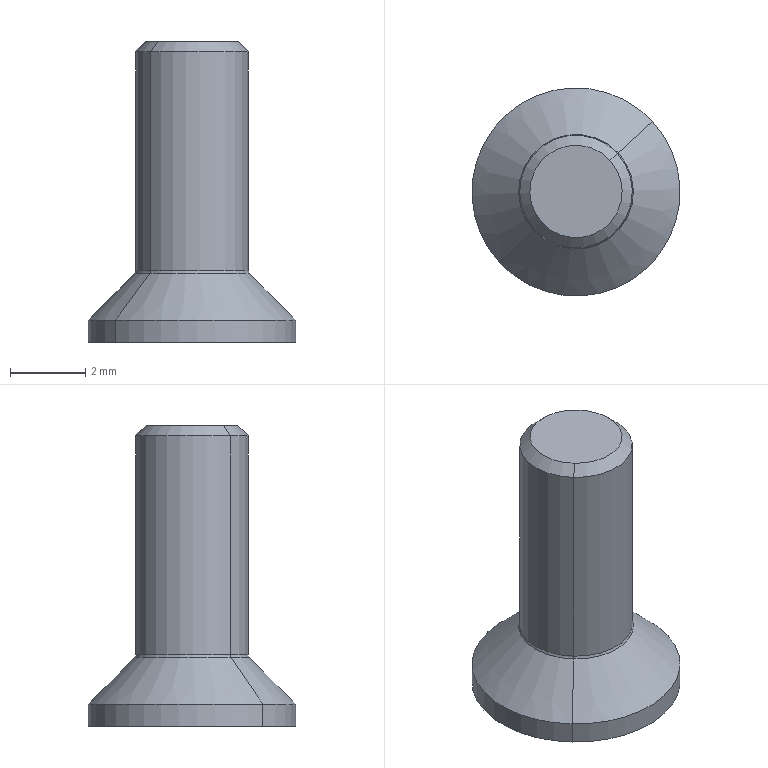Component | SolidWorks | V1ZHXTRR60SecondarySB1-1_v1ZHXTHexagon socket countersunk head screws GB_GB_FASTENER_SCREWS_HSCHS M3X8-N_1SB1-1 | 1 solid | 26 faces | box 5.54 x 5.54 x 8 mm | volume 72 mm3 | plane 14 | cone 6 | cylinder 4 | spline 2 | commonest cylinder face diameters 3 x2 5.54 x2
STEP:
#1=COLOUR_RGB('',0.7922,0.8196,0.9333);
#2=FILL_AREA_STYLE_COLOUR('',#1);
#3=FILL_AREA_STYLE('',(#2));
#4=SURFACE_STYLE_FILL_AREA(#3);
#5=SURFACE_SIDE_STYLE('',(#4));
#6=SURFACE_STYLE_USAGE(.BOTH.,#5);
#7=PRESENTATION_STYLE_ASSIGNMENT((#6));
#8=CARTESIAN_POINT('',(9.394,-8.991,18.832));
#9=VERTEX_POINT('',#8);
#10=CARTESIAN_POINT('',(9.307,-9.071,18.832));
#11=VERTEX_POINT('',#10);
#12=CARTESIAN_POINT('',(9.35,-9.031,18.832));
#13=DIRECTION('',(0.,-0.,1.));
#14=DIRECTION('',(-0.7334,-0.6798,-0.));
#15=AXIS2_PLACEMENT_3D('',#12,#13,#14);
#16=CIRCLE('',#15,0.05906);
#17=EDGE_CURVE('',#9,#11,#16,.T.);
#18=ORIENTED_EDGE('',*,*,#17,.F.);
#19=CARTESIAN_POINT('',(9.394,-8.99,18.83));
#20=VERTEX_POINT('',#19);
#21=CARTESIAN_POINT('',(9.396,-8.988,18.832));
#22=DIRECTION('',(0.6798,-0.7334,-0.));
#23=DIRECTION('',(0.7334,0.6798,0.));
#24=AXIS2_PLACEMENT_3D('',#21,#22,#23);
#25=CIRCLE('',#24,0.003937);
#26=EDGE_CURVE('',#9,#20,#25,.T.);
#27=ORIENTED_EDGE('',*,*,#26,.T.);
#28=CARTESIAN_POINT('',(9.306,-9.072,18.83));
#29=VERTEX_POINT('',#28);
#30=CARTESIAN_POINT('',(9.35,-9.031,18.83));
#31=DIRECTION('',(-0.,0.,-1.));
#32=DIRECTION('',(-0.7334,-0.6798,-0.));
#33=AXIS2_PLACEMENT_3D('',#30,#31,#32);
#34=CIRCLE('',#33,0.06021);
#35=EDGE_CURVE('',#29,#20,#34,.T.);
#36=ORIENTED_EDGE('',*,*,#35,.F.);
#37=CARTESIAN_POINT('',(9.304,-9.074,18.832));
#38=DIRECTION('',(-0.6798,0.7334,0.));
#39=DIRECTION('',(-0.7334,-0.6798,-0.));
#40=AXIS2_PLACEMENT_3D('',#37,#38,#39);
#41=CIRCLE('',#40,0.003937);
#42=EDGE_CURVE('',#11,#29,#41,.T.);
#43=ORIENTED_EDGE('',*,*,#42,.F.);
#44=EDGE_LOOP('',(#18,#27,#36,#43));
#45=FACE_OUTER_BOUND('',#44,.T.);
#46=CARTESIAN_POINT('',(9.307,-9.071,18.832));
#47=CARTESIAN_POINT('',(9.283,-9.046,18.832));
#48=CARTESIAN_POINT('',(9.285,-9.011,18.832));
#49=CARTESIAN_POINT('',(9.31,-8.988,18.832));
#50=CARTESIAN_POINT('',(9.336,-8.964,18.832));
#51=CARTESIAN_POINT('',(9.37,-8.966,18.832));
#52=CARTESIAN_POINT('',(9.394,-8.991,18.832));
#53=CARTESIAN_POINT('',(9.307,-9.071,18.831));
#54=CARTESIAN_POINT('',(9.283,-9.046,18.831));
#55=CARTESIAN_POINT('',(9.285,-9.011,18.831));
#56=CARTESIAN_POINT('',(9.31,-8.988,18.831));
#57=CARTESIAN_POINT('',(9.336,-8.964,18.831));
#58=CARTESIAN_POINT('',(9.37,-8.966,18.831));
#59=CARTESIAN_POINT('',(9.394,-8.991,18.831));
#60=CARTESIAN_POINT('',(9.307,-9.071,18.83));
#61=CARTESIAN_POINT('',(9.283,-9.046,18.83));
#62=CARTESIAN_POINT('',(9.284,-9.011,18.83));
#63=CARTESIAN_POINT('',(9.31,-8.987,18.83));
#64=CARTESIAN_POINT('',(9.335,-8.964,18.83));
#65=CARTESIAN_POINT('',(9.37,-8.965,18.83));
#66=CARTESIAN_POINT('',(9.394,-8.991,18.83));
#67=CARTESIAN_POINT('',(9.306,-9.072,18.83));
#68=CARTESIAN_POINT('',(9.282,-9.046,18.83));
#69=CARTESIAN_POINT('',(9.283,-9.011,18.83));
#70=CARTESIAN_POINT('',(9.309,-8.987,18.83));
#71=CARTESIAN_POINT('',(9.335,-8.963,18.83));
#72=CARTESIAN_POINT('',(9.37,-8.964,18.83));
#73=CARTESIAN_POINT('',(9.394,-8.99,18.83));
#74=(BOUNDED_SURFACE()B_SPLINE_SURFACE(3,3,((#46,#47,#48,#49,#50,#51,#52),(#53,#54,#55,#56,#57,#58,#59),(#60,#61,#62,#63,#64,#65,#66),(#67,#68,#69,#70,#71,#72,#73)),.UNSPECIFIED.,.F.,.F.,.F.)B_SPLINE_SURFACE_WITH_KNOTS((4,4),(4,3,4),(0.,1.),(0.,0.5,1.),.UNSPECIFIED.)GEOMETRIC_REPRESENTATION_ITEM()RATIONAL_B_SPLINE_SURFACE(((1.,0.8047,0.8047,1.,0.8047,0.8047,1.),(0.9493,0.7639,0.7639,0.9493,0.7639,0.7639,0.9493),(0.9493,0.7639,0.7639,0.9493,0.7639,0.7639,0.9493),(1.,0.8047,0.8047,1.,0.8047,0.8047,1.)))REPRESENTATION_ITEM('')SURFACE());
#75=ADVANCED_FACE('',(#45),#74,.F.);
#76=CARTESIAN_POINT('',(9.307,-9.071,19.062));
#77=VERTEX_POINT('',#76);
#78=CARTESIAN_POINT('',(9.394,-8.991,19.062));
#79=VERTEX_POINT('',#78);
#80=CARTESIAN_POINT('',(9.35,-9.031,19.062));
#81=DIRECTION('',(-0.,0.,-1.));
#82=DIRECTION('',(-0.7334,-0.6798,-0.));
#83=AXIS2_PLACEMENT_3D('',#80,#81,#82);
#84=CIRCLE('',#83,0.05906);
#85=EDGE_CURVE('',#77,#79,#84,.T.);
#86=ORIENTED_EDGE('',*,*,#85,.T.);
#87=CARTESIAN_POINT('',(9.394,-8.991,18.734));
#88=DIRECTION('',(-0.,0.,-1.));
#89=VECTOR('',#88,39.37);
#90=LINE('',#87,#89);
#91=EDGE_CURVE('',#79,#9,#90,.T.);
#92=ORIENTED_EDGE('',*,*,#91,.T.);
#93=ORIENTED_EDGE('',*,*,#17,.T.);
#94=CARTESIAN_POINT('',(9.307,-9.071,18.734));
#95=DIRECTION('',(-0.,0.,-1.));
#96=VECTOR('',#95,39.37);
#97=LINE('',#94,#96);
#98=EDGE_CURVE('',#77,#11,#97,.T.);
#99=ORIENTED_EDGE('',*,*,#98,.F.);
#100=EDGE_LOOP('',(#86,#92,#93,#99));
#101=FACE_OUTER_BOUND('',#100,.T.);
#102=CARTESIAN_POINT('',(9.35,-9.031,18.734));
#103=DIRECTION('',(-0.,0.,-1.));
#104=DIRECTION('',(-0.7334,-0.6798,-0.));
#105=AXIS2_PLACEMENT_3D('',#102,#103,#104);
#106=CYLINDRICAL_SURFACE('',#105,0.05906);
#107=ADVANCED_FACE('',(#101),#106,.T.);
#108=CARTESIAN_POINT('',(9.315,-9.064,19.072));
#109=VERTEX_POINT('',#108);
#110=CARTESIAN_POINT('',(9.386,-8.998,19.072));
#111=VERTEX_POINT('',#110);
#112=CARTESIAN_POINT('',(9.35,-9.031,19.072));
#113=DIRECTION('',(-0.,0.,-1.));
#114=DIRECTION('',(-0.7334,-0.6798,-0.));
#115=AXIS2_PLACEMENT_3D('',#112,#113,#114);
#116=CIRCLE('',#115,0.04841);
#117=EDGE_CURVE('',#109,#111,#116,.T.);
#118=ORIENTED_EDGE('',*,*,#117,.T.);
#119=CARTESIAN_POINT('',(9.394,-8.991,19.062));
#120=DIRECTION('',(0.5186,0.4807,-0.7071));
#121=VECTOR('',#120,39.37);
#122=LINE('',#119,#121);
#123=EDGE_CURVE('',#111,#79,#122,.T.);
#124=ORIENTED_EDGE('',*,*,#123,.T.);
#125=ORIENTED_EDGE('',*,*,#85,.F.);
#126=CARTESIAN_POINT('',(9.307,-9.071,19.062));
#127=DIRECTION('',(-0.5186,-0.4807,-0.7071));
#128=VECTOR('',#127,39.37);
#129=LINE('',#126,#128);
#130=EDGE_CURVE('',#109,#77,#129,.T.);
#131=ORIENTED_EDGE('',*,*,#130,.F.);
#132=EDGE_LOOP('',(#118,#124,#125,#131));
#133=FACE_OUTER_BOUND('',#132,.T.);
#134=CARTESIAN_POINT('',(9.35,-9.031,19.062));
#135=DIRECTION('',(-0.,0.,-1.));
#136=DIRECTION('',(-0.7334,-0.6798,-0.));
#137=AXIS2_PLACEMENT_3D('',#134,#135,#136);
#138=CONICAL_SURFACE('',#137,0.05906,0.7854);
#139=ADVANCED_FACE('',(#133),#138,.T.);
#140=ORIENTED_EDGE('',*,*,#35,.T.);
#141=CARTESIAN_POINT('',(9.43,-8.957,18.781));
#142=VERTEX_POINT('',#141);
#143=CARTESIAN_POINT('',(9.43,-8.957,18.781));
#144=DIRECTION('',(0.5186,0.4807,-0.7071));
#145=VECTOR('',#144,39.37);
#146=LINE('',#143,#145);
#147=EDGE_CURVE('',#20,#142,#146,.T.);
#148=ORIENTED_EDGE('',*,*,#147,.T.);
#149=CARTESIAN_POINT('',(9.27,-9.105,18.781));
#150=VERTEX_POINT('',#149);
#151=CARTESIAN_POINT('',(9.35,-9.031,18.781));
#152=DIRECTION('',(0.,-0.,1.));
#153=DIRECTION('',(-0.7334,-0.6798,-0.));
#154=AXIS2_PLACEMENT_3D('',#151,#152,#153);
#155=CIRCLE('',#154,0.1091);
#156=EDGE_CURVE('',#142,#150,#155,.T.);
#157=ORIENTED_EDGE('',*,*,#156,.T.);
#158=CARTESIAN_POINT('',(9.27,-9.105,18.781));
#159=DIRECTION('',(-0.5186,-0.4807,-0.7071));
#160=VECTOR('',#159,39.37);
#161=LINE('',#158,#160);
#162=EDGE_CURVE('',#29,#150,#161,.T.);
#163=ORIENTED_EDGE('',*,*,#162,.F.);
#164=EDGE_LOOP('',(#140,#148,#157,#163));
#165=FACE_OUTER_BOUND('',#164,.T.);
#166=CARTESIAN_POINT('',(9.35,-9.031,18.781));
#167=DIRECTION('',(-0.,0.,-1.));
#168=DIRECTION('',(-0.7334,-0.6798,-0.));
#169=AXIS2_PLACEMENT_3D('',#166,#167,#168);
#170=CONICAL_SURFACE('',#169,0.1091,0.7854);
#171=ADVANCED_FACE('',(#165),#170,.T.);
#172=CARTESIAN_POINT('',(9.43,-8.957,18.757));
#173=VERTEX_POINT('',#172);
#174=CARTESIAN_POINT('',(9.27,-9.105,18.757));
#175=VERTEX_POINT('',#174);
#176=CARTESIAN_POINT('',(9.35,-9.031,18.757));
#177=DIRECTION('',(0.,-0.,1.));
#178=DIRECTION('',(0.7334,0.6798,0.));
#179=AXIS2_PLACEMENT_3D('',#176,#177,#178);
#180=CIRCLE('',#179,0.1091);
#181=EDGE_CURVE('',#173,#175,#180,.T.);
#182=ORIENTED_EDGE('',*,*,#181,.T.);
#183=CARTESIAN_POINT('',(9.27,-9.105,19.224));
#184=DIRECTION('',(0.,-0.,1.));
#185=VECTOR('',#184,39.37);
#186=LINE('',#183,#185);
#187=EDGE_CURVE('',#175,#150,#186,.T.);
#188=ORIENTED_EDGE('',*,*,#187,.T.);
#189=ORIENTED_EDGE('',*,*,#156,.F.);
#190=CARTESIAN_POINT('',(9.43,-8.957,19.224));
#191=DIRECTION('',(0.,-0.,1.));
#192=VECTOR('',#191,39.37);
#193=LINE('',#190,#192);
#194=EDGE_CURVE('',#173,#142,#193,.T.);
#195=ORIENTED_EDGE('',*,*,#194,.F.);
#196=EDGE_LOOP('',(#182,#188,#189,#195));
#197=FACE_OUTER_BOUND('',#196,.T.);
#198=CARTESIAN_POINT('',(9.35,-9.031,19.224));
#199=DIRECTION('',(0.,-0.,1.));
#200=DIRECTION('',(0.7334,0.6798,0.));
#201=AXIS2_PLACEMENT_3D('',#198,#199,#200);
#202=CYLINDRICAL_SURFACE('',#201,0.1091);
#203=ADVANCED_FACE('',(#197),#202,.T.);
#204=CARTESIAN_POINT('',(9.35,-9.031,18.823));
#205=VERTEX_POINT('',#204);
#206=CARTESIAN_POINT('',(9.321,-9.058,18.801));
#207=VERTEX_POINT('',#206);
#208=CARTESIAN_POINT('',(9.321,-9.058,18.801));
#209=DIRECTION('',(-0.6351,-0.5888,-0.5));
#210=VECTOR('',#209,39.37);
#211=LINE('',#208,#210);
#212=EDGE_CURVE('',#205,#207,#211,.T.);
#213=ORIENTED_EDGE('',*,*,#212,.F.);
#214=CARTESIAN_POINT('',(9.379,-9.004,18.801));
#215=VERTEX_POINT('',#214);
#216=CARTESIAN_POINT('',(9.379,-9.004,18.801));
#217=DIRECTION('',(0.6351,0.5888,-0.5));
#218=VECTOR('',#217,39.37);
#219=LINE('',#216,#218);
#220=EDGE_CURVE('',#205,#215,#219,.T.);
#221=ORIENTED_EDGE('',*,*,#220,.T.);
#222=CARTESIAN_POINT('',(9.389,-9.022,18.801));
#223=VERTEX_POINT('',#222);
#224=CARTESIAN_POINT('',(9.35,-9.031,18.801));
#225=DIRECTION('',(-0.,0.,-1.));
#226=DIRECTION('',(-0.7334,-0.6798,-0.));
#227=AXIS2_PLACEMENT_3D('',#224,#225,#226);
#228=CIRCLE('',#227,0.03937);
#229=EDGE_CURVE('',#215,#223,#228,.T.);
#230=ORIENTED_EDGE('',*,*,#229,.T.);
#231=CARTESIAN_POINT('',(9.377,-9.06,18.801));
#232=VERTEX_POINT('',#231);
#233=CARTESIAN_POINT('',(9.35,-9.031,18.801));
#234=DIRECTION('',(-0.,0.,-1.));
#235=DIRECTION('',(-0.7334,-0.6798,-0.));
#236=AXIS2_PLACEMENT_3D('',#233,#234,#235);
#237=CIRCLE('',#236,0.03937);
#238=EDGE_CURVE('',#223,#232,#237,.T.);
#239=ORIENTED_EDGE('',*,*,#238,.T.);
#240=CARTESIAN_POINT('',(9.339,-9.069,18.801));
#241=VERTEX_POINT('',#240);
#242=CARTESIAN_POINT('',(9.35,-9.031,18.801));
#243=DIRECTION('',(-0.,0.,-1.));
#244=DIRECTION('',(-0.7334,-0.6798,-0.));
#245=AXIS2_PLACEMENT_3D('',#242,#243,#244);
#246=CIRCLE('',#245,0.03937);
#247=EDGE_CURVE('',#232,#241,#246,.T.);
#248=ORIENTED_EDGE('',*,*,#247,.T.);
#249=CARTESIAN_POINT('',(9.35,-9.031,18.801));
#250=DIRECTION('',(-0.,0.,-1.));
#251=DIRECTION('',(-0.7334,-0.6798,-0.));
#252=AXIS2_PLACEMENT_3D('',#249,#250,#251);
#253=CIRCLE('',#252,0.03937);
#254=EDGE_CURVE('',#241,#207,#253,.T.);
#255=ORIENTED_EDGE('',*,*,#254,.T.);
#256=EDGE_LOOP('',(#213,#221,#230,#239,#248,#255));
#257=FACE_OUTER_BOUND('',#256,.T.);
#258=CARTESIAN_POINT('',(9.35,-9.031,18.801));
#259=DIRECTION('',(-0.,0.,-1.));
#260=DIRECTION('',(-0.7334,-0.6798,-0.));
#261=AXIS2_PLACEMENT_3D('',#258,#259,#260);
#262=CONICAL_SURFACE('',#261,0.03937,1.047);
#263=ADVANCED_FACE('',(#257),#262,.F.);
#264=ORIENTED_EDGE('',*,*,#91,.F.);
#265=CARTESIAN_POINT('',(9.35,-9.031,19.062));
#266=DIRECTION('',(-0.,0.,-1.));
#267=DIRECTION('',(-0.7334,-0.6798,-0.));
#268=AXIS2_PLACEMENT_3D('',#265,#266,#267);
#269=CIRCLE('',#268,0.05906);
#270=EDGE_CURVE('',#79,#77,#269,.T.);
#271=ORIENTED_EDGE('',*,*,#270,.T.);
#272=ORIENTED_EDGE('',*,*,#98,.T.);
#273=CARTESIAN_POINT('',(9.35,-9.031,18.832));
#274=DIRECTION('',(0.,-0.,1.));
#275=DIRECTION('',(-0.7334,-0.6798,-0.));
#276=AXIS2_PLACEMENT_3D('',#273,#274,#275);
#277=CIRCLE('',#276,0.05906);
#278=EDGE_CURVE('',#11,#9,#277,.T.);
#279=ORIENTED_EDGE('',*,*,#278,.T.);
#280=EDGE_LOOP('',(#264,#271,#272,#279));
#281=FACE_OUTER_BOUND('',#280,.T.);
#282=CARTESIAN_POINT('',(9.35,-9.031,18.734));
#283=DIRECTION('',(-0.,0.,-1.));
#284=DIRECTION('',(-0.7334,-0.6798,-0.));
#285=AXIS2_PLACEMENT_3D('',#282,#283,#284);
#286=CYLINDRICAL_SURFACE('',#285,0.05906);
#287=ADVANCED_FACE('',(#281),#286,.T.);
#288=ORIENTED_EDGE('',*,*,#26,.F.);
#289=ORIENTED_EDGE('',*,*,#278,.F.);
#290=ORIENTED_EDGE('',*,*,#42,.T.);
#291=CARTESIAN_POINT('',(9.35,-9.031,18.83));
#292=DIRECTION('',(-0.,0.,-1.));
#293=DIRECTION('',(-0.7334,-0.6798,-0.));
#294=AXIS2_PLACEMENT_3D('',#291,#292,#293);
#295=CIRCLE('',#294,0.06021);
#296=EDGE_CURVE('',#20,#29,#295,.T.);
#297=ORIENTED_EDGE('',*,*,#296,.F.);
#298=EDGE_LOOP('',(#288,#289,#290,#297));
#299=FACE_OUTER_BOUND('',#298,.T.);
#300=CARTESIAN_POINT('',(9.394,-8.991,18.832));
#301=CARTESIAN_POINT('',(9.474,-9.078,18.832));
#302=CARTESIAN_POINT('',(9.387,-9.158,18.832));
#303=CARTESIAN_POINT('',(9.307,-9.071,18.832));
#304=CARTESIAN_POINT('',(9.394,-8.991,18.831));
#305=CARTESIAN_POINT('',(9.474,-9.078,18.831));
#306=CARTESIAN_POINT('',(9.387,-9.158,18.831));
#307=CARTESIAN_POINT('',(9.307,-9.071,18.831));
#308=CARTESIAN_POINT('',(9.394,-8.991,18.83));
#309=CARTESIAN_POINT('',(9.475,-9.078,18.83));
#310=CARTESIAN_POINT('',(9.388,-9.159,18.83));
#311=CARTESIAN_POINT('',(9.307,-9.071,18.83));
#312=CARTESIAN_POINT('',(9.394,-8.99,18.83));
#313=CARTESIAN_POINT('',(9.476,-9.078,18.83));
#314=CARTESIAN_POINT('',(9.388,-9.16,18.83));
#315=CARTESIAN_POINT('',(9.306,-9.072,18.83));
#316=(BOUNDED_SURFACE()B_SPLINE_SURFACE(3,3,((#300,#301,#302,#303),(#304,#305,#306,#307),(#308,#309,#310,#311),(#312,#313,#314,#315)),.UNSPECIFIED.,.F.,.F.,.F.)B_SPLINE_SURFACE_WITH_KNOTS((4,4),(4,4),(0.,1.),(0.,1.),.UNSPECIFIED.)GEOMETRIC_REPRESENTATION_ITEM()RATIONAL_B_SPLINE_SURFACE(((1.,0.3333,0.3333,1.),(0.9493,0.3164,0.3164,0.9493),(0.9493,0.3164,0.3164,0.9493),(1.,0.3333,0.3333,1.)))REPRESENTATION_ITEM('')SURFACE());
#317=ADVANCED_FACE('',(#299),#316,.F.);
#318=ORIENTED_EDGE('',*,*,#123,.F.);
#319=CARTESIAN_POINT('',(9.35,-9.031,19.072));
#320=DIRECTION('',(-0.,0.,-1.));
#321=DIRECTION('',(-0.7334,-0.6798,-0.));
#322=AXIS2_PLACEMENT_3D('',#319,#320,#321);
#323=CIRCLE('',#322,0.04841);
#324=EDGE_CURVE('',#111,#109,#323,.T.);
#325=ORIENTED_EDGE('',*,*,#324,.T.);
#326=ORIENTED_EDGE('',*,*,#130,.T.);
#327=ORIENTED_EDGE('',*,*,#270,.F.);
#328=EDGE_LOOP('',(#318,#325,#326,#327));
#329=FACE_OUTER_BOUND('',#328,.T.);
#330=CARTESIAN_POINT('',(9.35,-9.031,19.062));
#331=DIRECTION('',(-0.,0.,-1.));
#332=DIRECTION('',(-0.7334,-0.6798,-0.));
#333=AXIS2_PLACEMENT_3D('',#330,#331,#332);
#334=CONICAL_SURFACE('',#333,0.05906,0.7854);
#335=ADVANCED_FACE('',(#329),#334,.T.);
#336=ORIENTED_EDGE('',*,*,#147,.F.);
#337=ORIENTED_EDGE('',*,*,#296,.T.);
#338=ORIENTED_EDGE('',*,*,#162,.T.);
#339=CARTESIAN_POINT('',(9.35,-9.031,18.781));
#340=DIRECTION('',(0.,-0.,1.));
#341=DIRECTION('',(-0.7334,-0.6798,-0.));
#342=AXIS2_PLACEMENT_3D('',#339,#340,#341);
#343=CIRCLE('',#342,0.1091);
#344=EDGE_CURVE('',#150,#142,#343,.T.);
#345=ORIENTED_EDGE('',*,*,#344,.T.);
#346=EDGE_LOOP('',(#336,#337,#338,#345));
#347=FACE_OUTER_BOUND('',#346,.T.);
#348=CARTESIAN_POINT('',(9.35,-9.031,18.781));
#349=DIRECTION('',(-0.,0.,-1.));
#350=DIRECTION('',(-0.7334,-0.6798,-0.));
#351=AXIS2_PLACEMENT_3D('',#348,#349,#350);
#352=CONICAL_SURFACE('',#351,0.1091,0.7854);
#353=ADVANCED_FACE('',(#347),#352,.T.);
#354=ORIENTED_EDGE('',*,*,#117,.F.);
#355=ORIENTED_EDGE('',*,*,#324,.F.);
#356=EDGE_LOOP('',(#354,#355));
#357=FACE_OUTER_BOUND('',#356,.T.);
#358=CARTESIAN_POINT('',(9.31,-8.988,19.072));
#359=DIRECTION('',(-0.,0.,-1.));
#360=DIRECTION('',(-0.7334,-0.6798,-0.));
#361=AXIS2_PLACEMENT_3D('',#358,#359,#360);
#362=PLANE('',#361);
#363=ADVANCED_FACE('',(#357),#362,.F.);
#364=ORIENTED_EDGE('',*,*,#187,.F.);
#365=CARTESIAN_POINT('',(9.35,-9.031,18.757));
#366=DIRECTION('',(0.,-0.,1.));
#367=DIRECTION('',(0.7334,0.6798,0.));
#368=AXIS2_PLACEMENT_3D('',#365,#366,#367);
#369=CIRCLE('',#368,0.1091);
#370=EDGE_CURVE('',#175,#173,#369,.T.);
#371=ORIENTED_EDGE('',*,*,#370,.T.);
#372=ORIENTED_EDGE('',*,*,#194,.T.);
#373=ORIENTED_EDGE('',*,*,#344,.F.);
#374=EDGE_LOOP('',(#364,#371,#372,#373));
#375=FACE_OUTER_BOUND('',#374,.T.);
#376=CARTESIAN_POINT('',(9.35,-9.031,19.224));
#377=DIRECTION('',(0.,-0.,1.));
#378=DIRECTION('',(0.7334,0.6798,0.));
#379=AXIS2_PLACEMENT_3D('',#376,#377,#378);
#380=CYLINDRICAL_SURFACE('',#379,0.1091);
#381=ADVANCED_FACE('',(#375),#380,.T.);
#382=CARTESIAN_POINT('',(9.34,-8.987,18.757));
#383=VERTEX_POINT('',#382);
#384=CARTESIAN_POINT('',(9.384,-9.,18.757));
#385=VERTEX_POINT('',#384);
#386=CARTESIAN_POINT('',(9.34,-8.987,18.757));
#387=DIRECTION('',(0.9554,-0.2952,-0.));
#388=VECTOR('',#387,39.37);
#389=LINE('',#386,#388);
#390=EDGE_CURVE('',#383,#385,#389,.T.);
#391=ORIENTED_EDGE('',*,*,#390,.F.);
#392=CARTESIAN_POINT('',(9.307,-9.018,18.757));
#393=VERTEX_POINT('',#392);
#394=CARTESIAN_POINT('',(9.324,-9.002,18.757));
#395=DIRECTION('',(0.7334,0.6798,0.));
#396=VECTOR('',#395,39.37);
#397=LINE('',#394,#396);
#398=EDGE_CURVE('',#393,#383,#397,.T.);
#399=ORIENTED_EDGE('',*,*,#398,.F.);
#400=CARTESIAN_POINT('',(9.317,-9.062,18.757));
#401=VERTEX_POINT('',#400);
#402=CARTESIAN_POINT('',(9.317,-9.062,18.757));
#403=DIRECTION('',(-0.2221,0.975,0.));
#404=VECTOR('',#403,39.37);
#405=LINE('',#402,#404);
#406=EDGE_CURVE('',#401,#393,#405,.T.);
#407=ORIENTED_EDGE('',*,*,#406,.F.);
#408=CARTESIAN_POINT('',(9.36,-9.075,18.757));
#409=VERTEX_POINT('',#408);
#410=CARTESIAN_POINT('',(9.36,-9.075,18.757));
#411=DIRECTION('',(-0.9554,0.2952,0.));
#412=VECTOR('',#411,39.37);
#413=LINE('',#410,#412);
#414=EDGE_CURVE('',#409,#401,#413,.T.);
#415=ORIENTED_EDGE('',*,*,#414,.F.);
#416=CARTESIAN_POINT('',(9.394,-9.044,18.757));
#417=VERTEX_POINT('',#416);
#418=CARTESIAN_POINT('',(9.377,-9.06,18.757));
#419=DIRECTION('',(-0.7334,-0.6798,-0.));
#420=VECTOR('',#419,39.37);
#421=LINE('',#418,#420);
#422=EDGE_CURVE('',#417,#409,#421,.T.);
#423=ORIENTED_EDGE('',*,*,#422,.F.);
#424=CARTESIAN_POINT('',(9.384,-9.,18.757));
#425=DIRECTION('',(0.2221,-0.975,-0.));
#426=VECTOR('',#425,39.37);
#427=LINE('',#424,#426);
#428=EDGE_CURVE('',#385,#417,#427,.T.);
#429=ORIENTED_EDGE('',*,*,#428,.F.);
#430=EDGE_LOOP('',(#391,#399,#407,#415,#423,#429));
#431=FACE_BOUND('',#430,.T.);
#432=ORIENTED_EDGE('',*,*,#181,.F.);
#433=ORIENTED_EDGE('',*,*,#370,.F.);
#434=EDGE_LOOP('',(#432,#433));
#435=FACE_OUTER_BOUND('',#434,.T.);
#436=CARTESIAN_POINT('',(9.35,-9.031,18.757));
#437=DIRECTION('',(0.,-0.,1.));
#438=DIRECTION('',(0.7334,0.6798,0.));
#439=AXIS2_PLACEMENT_3D('',#436,#437,#438);
#440=PLANE('',#439);
#441=ADVANCED_FACE('',(#431,#435),#440,.F.);
#442=CARTESIAN_POINT('',(9.384,-9.,18.801));
#443=VERTEX_POINT('',#442);
#444=CARTESIAN_POINT('',(9.394,-9.044,18.801));
#445=DIRECTION('',(-0.2221,0.975,0.));
#446=VECTOR('',#445,39.37);
#447=LINE('',#444,#446);
#448=EDGE_CURVE('',#223,#443,#447,.T.);
#449=ORIENTED_EDGE('',*,*,#448,.T.);
#450=CARTESIAN_POINT('',(9.384,-9.,18.801));
#451=DIRECTION('',(-0.,0.,-1.));
#452=VECTOR('',#451,39.37);
#453=LINE('',#450,#452);
#454=EDGE_CURVE('',#443,#385,#453,.T.);
#455=ORIENTED_EDGE('',*,*,#454,.T.);
#456=ORIENTED_EDGE('',*,*,#428,.T.);
#457=CARTESIAN_POINT('',(9.394,-9.044,18.801));
#458=VERTEX_POINT('',#457);
#459=CARTESIAN_POINT('',(9.394,-9.044,18.801));
#460=DIRECTION('',(0.,-0.,1.));
#461=VECTOR('',#460,39.37);
#462=LINE('',#459,#461);
#463=EDGE_CURVE('',#417,#458,#462,.T.);
#464=ORIENTED_EDGE('',*,*,#463,.T.);
#465=CARTESIAN_POINT('',(9.394,-9.044,18.801));
#466=DIRECTION('',(-0.2221,0.975,0.));
#467=VECTOR('',#466,39.37);
#468=LINE('',#465,#467);
#469=EDGE_CURVE('',#458,#223,#468,.T.);
#470=ORIENTED_EDGE('',*,*,#469,.T.);
#471=EDGE_LOOP('',(#449,#455,#456,#464,#470));
#472=FACE_OUTER_BOUND('',#471,.T.);
#473=CARTESIAN_POINT('',(9.394,-9.044,18.801));
#474=DIRECTION('',(-0.975,-0.2221,-0.));
#475=DIRECTION('',(0.2221,-0.975,-0.));
#476=AXIS2_PLACEMENT_3D('',#473,#474,#475);
#477=PLANE('',#476);
#478=ADVANCED_FACE('',(#472),#477,.T.);
#479=CARTESIAN_POINT('',(9.362,-8.993,18.801));
#480=VERTEX_POINT('',#479);
#481=CARTESIAN_POINT('',(9.34,-8.987,18.801));
#482=VERTEX_POINT('',#481);
#483=CARTESIAN_POINT('',(9.384,-9.,18.801));
#484=DIRECTION('',(-0.9554,0.2952,0.));
#485=VECTOR('',#484,39.37);
#486=LINE('',#483,#485);
#487=EDGE_CURVE('',#480,#482,#486,.T.);
#488=ORIENTED_EDGE('',*,*,#487,.T.);
#489=CARTESIAN_POINT('',(9.34,-8.987,18.801));
#490=DIRECTION('',(-0.,0.,-1.));
#491=VECTOR('',#490,39.37);
#492=LINE('',#489,#491);
#493=EDGE_CURVE('',#482,#383,#492,.T.);
#494=ORIENTED_EDGE('',*,*,#493,.T.);
#495=ORIENTED_EDGE('',*,*,#390,.T.);
#496=ORIENTED_EDGE('',*,*,#454,.F.);
#497=CARTESIAN_POINT('',(9.384,-9.,18.801));
#498=DIRECTION('',(-0.9554,0.2952,0.));
#499=VECTOR('',#498,39.37);
#500=LINE('',#497,#499);
#501=EDGE_CURVE('',#443,#480,#500,.T.);
#502=ORIENTED_EDGE('',*,*,#501,.T.);
#503=EDGE_LOOP('',(#488,#494,#495,#496,#502));
#504=FACE_OUTER_BOUND('',#503,.T.);
#505=CARTESIAN_POINT('',(9.384,-9.,18.801));
#506=DIRECTION('',(-0.2952,-0.9554,-0.));
#507=DIRECTION('',(0.9554,-0.2952,-0.));
#508=AXIS2_PLACEMENT_3D('',#505,#506,#507);
#509=PLANE('',#508);
#510=ADVANCED_FACE('',(#504),#509,.T.);
#511=CARTESIAN_POINT('',(9.324,-9.002,18.801));
#512=VERTEX_POINT('',#511);
#513=CARTESIAN_POINT('',(9.307,-9.018,18.801));
#514=VERTEX_POINT('',#513);
#515=CARTESIAN_POINT('',(9.34,-8.987,18.801));
#516=DIRECTION('',(-0.7334,-0.6798,-0.));
#517=VECTOR('',#516,39.37);
#518=LINE('',#515,#517);
#519=EDGE_CURVE('',#512,#514,#518,.T.);
#520=ORIENTED_EDGE('',*,*,#519,.T.);
#521=CARTESIAN_POINT('',(9.307,-9.018,18.801));
#522=DIRECTION('',(-0.,0.,-1.));
#523=VECTOR('',#522,39.37);
#524=LINE('',#521,#523);
#525=EDGE_CURVE('',#514,#393,#524,.T.);
#526=ORIENTED_EDGE('',*,*,#525,.T.);
#527=ORIENTED_EDGE('',*,*,#398,.T.);
#528=ORIENTED_EDGE('',*,*,#493,.F.);
#529=CARTESIAN_POINT('',(9.34,-8.987,18.801));
#530=DIRECTION('',(-0.7334,-0.6798,-0.));
#531=VECTOR('',#530,39.37);
#532=LINE('',#529,#531);
#533=EDGE_CURVE('',#482,#512,#532,.T.);
#534=ORIENTED_EDGE('',*,*,#533,.T.);
#535=EDGE_LOOP('',(#520,#526,#527,#528,#534));
#536=FACE_OUTER_BOUND('',#535,.T.);
#537=CARTESIAN_POINT('',(9.34,-8.987,18.801));
#538=DIRECTION('',(0.6798,-0.7334,-0.));
#539=DIRECTION('',(0.7334,0.6798,0.));
#540=AXIS2_PLACEMENT_3D('',#537,#538,#539);
#541=PLANE('',#540);
#542=ADVANCED_FACE('',(#536),#541,.T.);
#543=CARTESIAN_POINT('',(9.312,-9.04,18.801));
#544=VERTEX_POINT('',#543);
#545=CARTESIAN_POINT('',(9.317,-9.062,18.801));
#546=VERTEX_POINT('',#545);
#547=CARTESIAN_POINT('',(9.307,-9.018,18.801));
#548=DIRECTION('',(0.2221,-0.975,-0.));
#549=VECTOR('',#548,39.37);
#550=LINE('',#547,#549);
#551=EDGE_CURVE('',#544,#546,#550,.T.);
#552=ORIENTED_EDGE('',*,*,#551,.T.);
#553=CARTESIAN_POINT('',(9.317,-9.062,18.801));
#554=DIRECTION('',(-0.,0.,-1.));
#555=VECTOR('',#554,39.37);
#556=LINE('',#553,#555);
#557=EDGE_CURVE('',#546,#401,#556,.T.);
#558=ORIENTED_EDGE('',*,*,#557,.T.);
#559=ORIENTED_EDGE('',*,*,#406,.T.);
#560=ORIENTED_EDGE('',*,*,#525,.F.);
#561=CARTESIAN_POINT('',(9.307,-9.018,18.801));
#562=DIRECTION('',(0.2221,-0.975,-0.));
#563=VECTOR('',#562,39.37);
#564=LINE('',#561,#563);
#565=EDGE_CURVE('',#514,#544,#564,.T.);
#566=ORIENTED_EDGE('',*,*,#565,.T.);
#567=EDGE_LOOP('',(#552,#558,#559,#560,#566));
#568=FACE_OUTER_BOUND('',#567,.T.);
#569=CARTESIAN_POINT('',(9.307,-9.018,18.801));
#570=DIRECTION('',(0.975,0.2221,0.));
#571=DIRECTION('',(-0.2221,0.975,0.));
#572=AXIS2_PLACEMENT_3D('',#569,#570,#571);
#573=PLANE('',#572);
#574=ADVANCED_FACE('',(#568),#573,.T.);
#575=CARTESIAN_POINT('',(9.36,-9.075,18.801));
#576=VERTEX_POINT('',#575);
#577=CARTESIAN_POINT('',(9.317,-9.062,18.801));
#578=DIRECTION('',(0.9554,-0.2952,-0.));
#579=VECTOR('',#578,39.37);
#580=LINE('',#577,#579);
#581=EDGE_CURVE('',#241,#576,#580,.T.);
#582=ORIENTED_EDGE('',*,*,#581,.T.);
#583=CARTESIAN_POINT('',(9.36,-9.075,18.801));
#584=DIRECTION('',(-0.,0.,-1.));
#585=VECTOR('',#584,39.37);
#586=LINE('',#583,#585);
#587=EDGE_CURVE('',#576,#409,#586,.T.);
#588=ORIENTED_EDGE('',*,*,#587,.T.);
#589=ORIENTED_EDGE('',*,*,#414,.T.);
#590=ORIENTED_EDGE('',*,*,#557,.F.);
#591=CARTESIAN_POINT('',(9.317,-9.062,18.801));
#592=DIRECTION('',(0.9554,-0.2952,-0.));
#593=VECTOR('',#592,39.37);
#594=LINE('',#591,#593);
#595=EDGE_CURVE('',#546,#241,#594,.T.);
#596=ORIENTED_EDGE('',*,*,#595,.T.);
#597=EDGE_LOOP('',(#582,#588,#589,#590,#596));
#598=FACE_OUTER_BOUND('',#597,.T.);
#599=CARTESIAN_POINT('',(9.317,-9.062,18.801));
#600=DIRECTION('',(0.2952,0.9554,0.));
#601=DIRECTION('',(-0.9554,0.2952,0.));
#602=AXIS2_PLACEMENT_3D('',#599,#600,#601);
#603=PLANE('',#602);
#604=ADVANCED_FACE('',(#598),#603,.T.);
#605=CARTESIAN_POINT('',(9.36,-9.075,18.801));
#606=DIRECTION('',(0.7334,0.6798,0.));
#607=VECTOR('',#606,39.37);
#608=LINE('',#605,#607);
#609=EDGE_CURVE('',#232,#458,#608,.T.);
#610=ORIENTED_EDGE('',*,*,#609,.T.);
#611=ORIENTED_EDGE('',*,*,#463,.F.);
#612=ORIENTED_EDGE('',*,*,#422,.T.);
#613=ORIENTED_EDGE('',*,*,#587,.F.);
#614=CARTESIAN_POINT('',(9.36,-9.075,18.801));
#615=DIRECTION('',(0.7334,0.6798,0.));
#616=VECTOR('',#615,39.37);
#617=LINE('',#614,#616);
#618=EDGE_CURVE('',#576,#232,#617,.T.);
#619=ORIENTED_EDGE('',*,*,#618,.T.);
#620=EDGE_LOOP('',(#610,#611,#612,#613,#619));
#621=FACE_OUTER_BOUND('',#620,.T.);
#622=CARTESIAN_POINT('',(9.36,-9.075,18.801));
#623=DIRECTION('',(-0.6798,0.7334,0.));
#624=DIRECTION('',(-0.7334,-0.6798,-0.));
#625=AXIS2_PLACEMENT_3D('',#622,#623,#624);
#626=PLANE('',#625);
#627=ADVANCED_FACE('',(#621),#626,.T.);
#628=ORIENTED_EDGE('',*,*,#501,.F.);
#629=ORIENTED_EDGE('',*,*,#448,.F.);
#630=ORIENTED_EDGE('',*,*,#229,.F.);
#631=CARTESIAN_POINT('',(9.35,-9.031,18.801));
#632=DIRECTION('',(-0.,0.,-1.));
#633=DIRECTION('',(-0.7334,-0.6798,-0.));
#634=AXIS2_PLACEMENT_3D('',#631,#632,#633);
#635=CIRCLE('',#634,0.03937);
#636=EDGE_CURVE('',#480,#215,#635,.T.);
#637=ORIENTED_EDGE('',*,*,#636,.F.);
#638=EDGE_LOOP('',(#628,#629,#630,#637));
#639=FACE_OUTER_BOUND('',#638,.T.);
#640=CARTESIAN_POINT('',(9.384,-9.,18.801));
#641=DIRECTION('',(0.,-0.,1.));
#642=DIRECTION('',(0.7334,0.6798,0.));
#643=AXIS2_PLACEMENT_3D('',#640,#641,#642);
#644=PLANE('',#643);
#645=ADVANCED_FACE('',(#639),#644,.F.);
#646=ORIENTED_EDGE('',*,*,#469,.F.);
#647=ORIENTED_EDGE('',*,*,#609,.F.);
#648=ORIENTED_EDGE('',*,*,#238,.F.);
#649=EDGE_LOOP('',(#646,#647,#648));
#650=FACE_OUTER_BOUND('',#649,.T.);
#651=CARTESIAN_POINT('',(9.384,-9.,18.801));
#652=DIRECTION('',(0.,-0.,1.));
#653=DIRECTION('',(0.7334,0.6798,0.));
#654=AXIS2_PLACEMENT_3D('',#651,#652,#653);
#655=PLANE('',#654);
#656=ADVANCED_FACE('',(#650),#655,.F.);
#657=ORIENTED_EDGE('',*,*,#533,.F.);
#658=ORIENTED_EDGE('',*,*,#487,.F.);
#659=CARTESIAN_POINT('',(9.35,-9.031,18.801));
#660=DIRECTION('',(-0.,0.,-1.));
#661=DIRECTION('',(-0.7334,-0.6798,-0.));
#662=AXIS2_PLACEMENT_3D('',#659,#660,#661);
#663=CIRCLE('',#662,0.03937);
#664=EDGE_CURVE('',#512,#480,#663,.T.);
#665=ORIENTED_EDGE('',*,*,#664,.F.);
#666=EDGE_LOOP('',(#657,#658,#665));
#667=FACE_OUTER_BOUND('',#666,.T.);
#668=CARTESIAN_POINT('',(9.384,-9.,18.801));
#669=DIRECTION('',(0.,-0.,1.));
#670=DIRECTION('',(0.7334,0.6798,0.));
#671=AXIS2_PLACEMENT_3D('',#668,#669,#670);
#672=PLANE('',#671);
#673=ADVANCED_FACE('',(#667),#672,.F.);
#674=ORIENTED_EDGE('',*,*,#565,.F.);
#675=ORIENTED_EDGE('',*,*,#519,.F.);
#676=CARTESIAN_POINT('',(9.35,-9.031,18.801));
#677=DIRECTION('',(-0.,0.,-1.));
#678=DIRECTION('',(-0.7334,-0.6798,-0.));
#679=AXIS2_PLACEMENT_3D('',#676,#677,#678);
#680=CIRCLE('',#679,0.03937);
#681=EDGE_CURVE('',#544,#512,#680,.T.);
#682=ORIENTED_EDGE('',*,*,#681,.F.);
#683=EDGE_LOOP('',(#674,#675,#682));
#684=FACE_OUTER_BOUND('',#683,.T.);
#685=CARTESIAN_POINT('',(9.384,-9.,18.801));
#686=DIRECTION('',(0.,-0.,1.));
#687=DIRECTION('',(0.7334,0.6798,0.));
#688=AXIS2_PLACEMENT_3D('',#685,#686,#687);
#689=PLANE('',#688);
#690=ADVANCED_FACE('',(#684),#689,.F.);
#691=ORIENTED_EDGE('',*,*,#595,.F.);
#692=ORIENTED_EDGE('',*,*,#551,.F.);
#693=CARTESIAN_POINT('',(9.35,-9.031,18.801));
#694=DIRECTION('',(-0.,0.,-1.));
#695=DIRECTION('',(-0.7334,-0.6798,-0.));
#696=AXIS2_PLACEMENT_3D('',#693,#694,#695);
#697=CIRCLE('',#696,0.03937);
#698=EDGE_CURVE('',#207,#544,#697,.T.);
#699=ORIENTED_EDGE('',*,*,#698,.F.);
#700=ORIENTED_EDGE('',*,*,#254,.F.);
#701=EDGE_LOOP('',(#691,#692,#699,#700));
#702=FACE_OUTER_BOUND('',#701,.T.);
#703=CARTESIAN_POINT('',(9.384,-9.,18.801));
#704=DIRECTION('',(0.,-0.,1.));
#705=DIRECTION('',(0.7334,0.6798,0.));
#706=AXIS2_PLACEMENT_3D('',#703,#704,#705);
#707=PLANE('',#706);
#708=ADVANCED_FACE('',(#702),#707,.F.);
#709=ORIENTED_EDGE('',*,*,#618,.F.);
#710=ORIENTED_EDGE('',*,*,#581,.F.);
#711=ORIENTED_EDGE('',*,*,#247,.F.);
#712=EDGE_LOOP('',(#709,#710,#711));
#713=FACE_OUTER_BOUND('',#712,.T.);
#714=CARTESIAN_POINT('',(9.384,-9.,18.801));
#715=DIRECTION('',(0.,-0.,1.));
#716=DIRECTION('',(0.7334,0.6798,0.));
#717=AXIS2_PLACEMENT_3D('',#714,#715,#716);
#718=PLANE('',#717);
#719=ADVANCED_FACE('',(#713),#718,.F.);
#720=ORIENTED_EDGE('',*,*,#220,.F.);
#721=ORIENTED_EDGE('',*,*,#212,.T.);
#722=ORIENTED_EDGE('',*,*,#698,.T.);
#723=ORIENTED_EDGE('',*,*,#681,.T.);
#724=ORIENTED_EDGE('',*,*,#664,.T.);
#725=ORIENTED_EDGE('',*,*,#636,.T.);
#726=EDGE_LOOP('',(#720,#721,#722,#723,#724,#725));
#727=FACE_OUTER_BOUND('',#726,.T.);
#728=CARTESIAN_POINT('',(9.35,-9.031,18.801));
#729=DIRECTION('',(-0.,0.,-1.));
#730=DIRECTION('',(-0.7334,-0.6798,-0.));
#731=AXIS2_PLACEMENT_3D('',#728,#729,#730);
#732=CONICAL_SURFACE('',#731,0.03937,1.047);
#733=ADVANCED_FACE('',(#727),#732,.F.);
#734=CLOSED_SHELL('',(#75,#107,#139,#171,#203,#263,#287,#317,#335,#353,#363,#381,#441,#478,#510,#542,#574,#604,#627,#645,#656,#673,#690,#708,#719,#733));
#735=MANIFOLD_SOLID_BREP('',#734);
#736=STYLED_ITEM('',(#7),#735);
#737=PRESENTATION_LAYER_ASSIGNMENT('','',(#736));
#738=CARTESIAN_POINT('',(0.,0.,0.));
#739=DIRECTION('',(0.,0.,1.));
#740=DIRECTION('',(1.,0.,0.));
#741=AXIS2_PLACEMENT_3D('',#738,#739,#740);
#742=(LENGTH_UNIT()NAMED_UNIT(*)SI_UNIT($,.METRE.));
#743=LENGTH_MEASURE_WITH_UNIT(LENGTH_MEASURE(0.0254),#742);
#744=DIMENSIONAL_EXPONENTS(1.,0.,0.,0.,0.,0.,0.);
#745=(CONVERSION_BASED_UNIT('',#743)LENGTH_UNIT()NAMED_UNIT(#744));
#746=UNCERTAINTY_MEASURE_WITH_UNIT(LENGTH_MEASURE(0.00001),#745,'','');
#747=(NAMED_UNIT(*)PLANE_ANGLE_UNIT()SI_UNIT($,.RADIAN.));
#748=(NAMED_UNIT(*)SI_UNIT($,.STERADIAN.)SOLID_ANGLE_UNIT());
#749=(GEOMETRIC_REPRESENTATION_CONTEXT(3)GLOBAL_UNCERTAINTY_ASSIGNED_CONTEXT((#746))GLOBAL_UNIT_ASSIGNED_CONTEXT((#745,#747,#748))REPRESENTATION_CONTEXT('',''));
#750=ADVANCED_BREP_SHAPE_REPRESENTATION('',(#735,#741),#749);
#751=(LENGTH_UNIT()NAMED_UNIT(*)SI_UNIT($,.METRE.));
#752=LENGTH_MEASURE_WITH_UNIT(LENGTH_MEASURE(0.0254),#751);
#753=DIMENSIONAL_EXPONENTS(1.,0.,0.,0.,0.,0.,0.);
#754=(CONVERSION_BASED_UNIT('',#752)LENGTH_UNIT()NAMED_UNIT(#753));
#755=UNCERTAINTY_MEASURE_WITH_UNIT(LENGTH_MEASURE(0.00001),#754,'','');
#756=(NAMED_UNIT(*)PLANE_ANGLE_UNIT()SI_UNIT($,.RADIAN.));
#757=(NAMED_UNIT(*)SI_UNIT($,.STERADIAN.)SOLID_ANGLE_UNIT());
#758=(GEOMETRIC_REPRESENTATION_CONTEXT(3)GLOBAL_UNCERTAINTY_ASSIGNED_CONTEXT((#755))GLOBAL_UNIT_ASSIGNED_CONTEXT((#754,#756,#757))REPRESENTATION_CONTEXT('',''));
#759=MECHANICAL_DESIGN_GEOMETRIC_PRESENTATION_REPRESENTATION('',(#736),#758);